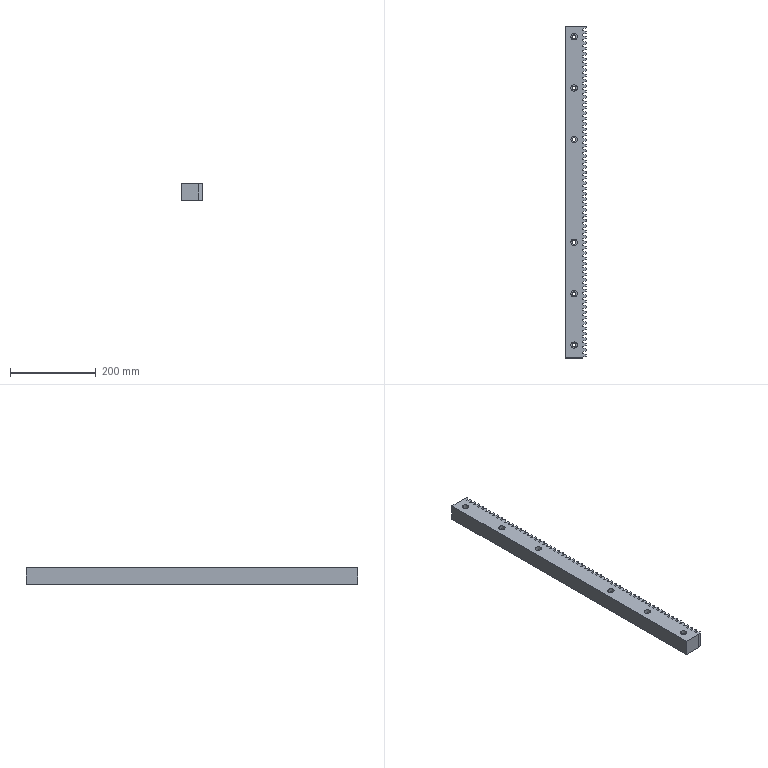Component | SolidWorks | DriveRackPart-1 | 1 solid | 283 faces | volume 1297926 mm3 | plane 259 | cylinder 24 | commonest cylinder face diameters 15 x12 9 x12